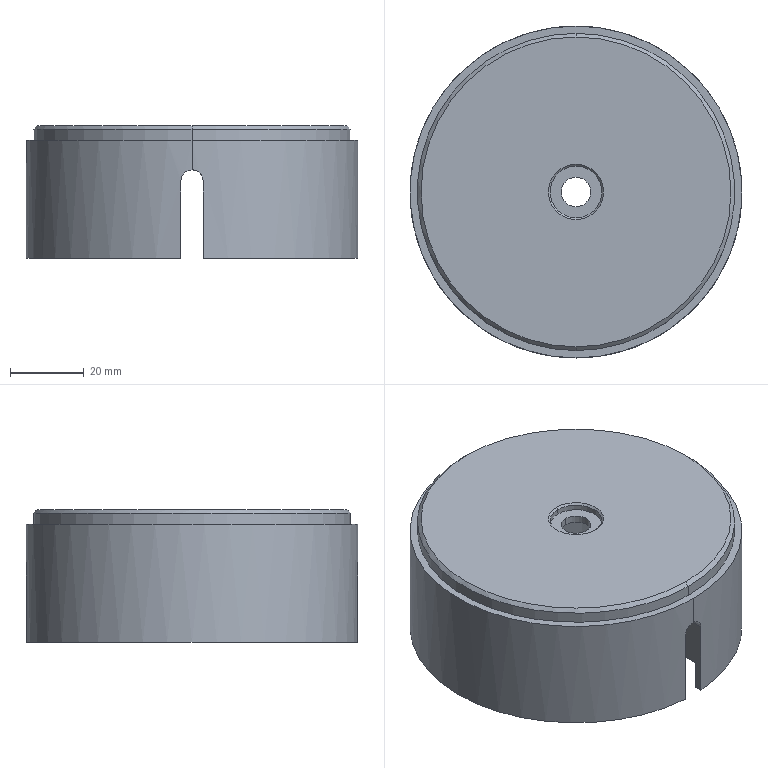Component | SolidWorks | GuideCover-1 | 1 solid | 32 faces | box 90 x 90 x 36 mm | volume 64020 mm3 | cylinder 14 | plane 12 | cone 4 | torus 2 | commonest cylinder face diameters 86 x4 14 x2 90 x2 8 x2 78 x2 6 x2
STEP:
#1=COLOUR_RGB('',0.7922,0.8196,0.9333);
#2=FILL_AREA_STYLE_COLOUR('',#1);
#3=FILL_AREA_STYLE('',(#2));
#4=SURFACE_STYLE_FILL_AREA(#3);
#5=SURFACE_SIDE_STYLE('',(#4));
#6=SURFACE_STYLE_USAGE(.BOTH.,#5);
#7=PRESENTATION_STYLE_ASSIGNMENT((#6));
#8=CARTESIAN_POINT('',(-0.6271,0.2087,2.579));
#9=VERTEX_POINT('',#8);
#10=CARTESIAN_POINT('',(-0.6271,-0.3425,2.579));
#11=VERTEX_POINT('',#10);
#12=CARTESIAN_POINT('',(-0.6271,-0.06694,2.579));
#13=DIRECTION('',(0.,0.,1.));
#14=DIRECTION('',(0.,-1.,0.));
#15=AXIS2_PLACEMENT_3D('',#12,#13,#14);
#16=CIRCLE('',#15,0.2756);
#17=EDGE_CURVE('',#9,#11,#16,.T.);
#18=ORIENTED_EDGE('',*,*,#17,.F.);
#19=CARTESIAN_POINT('',(-0.6271,0.2283,2.598));
#20=VERTEX_POINT('',#19);
#21=CARTESIAN_POINT('',(-0.6271,0.2087,2.579));
#22=DIRECTION('',(0.,0.7071,0.7071));
#23=VECTOR('',#22,39.37);
#24=LINE('',#21,#23);
#25=EDGE_CURVE('',#9,#20,#24,.T.);
#26=ORIENTED_EDGE('',*,*,#25,.T.);
#27=CARTESIAN_POINT('',(-0.6271,-0.3622,2.598));
#28=VERTEX_POINT('',#27);
#29=CARTESIAN_POINT('',(-0.6271,-0.06694,2.598));
#30=DIRECTION('',(0.,0.,-1.));
#31=DIRECTION('',(0.,-1.,0.));
#32=AXIS2_PLACEMENT_3D('',#29,#30,#31);
#33=CIRCLE('',#32,0.2953);
#34=EDGE_CURVE('',#28,#20,#33,.T.);
#35=ORIENTED_EDGE('',*,*,#34,.F.);
#36=CARTESIAN_POINT('',(-0.6271,-0.3425,2.579));
#37=DIRECTION('',(0.,-0.7071,0.7071));
#38=VECTOR('',#37,39.37);
#39=LINE('',#36,#38);
#40=EDGE_CURVE('',#11,#28,#39,.T.);
#41=ORIENTED_EDGE('',*,*,#40,.F.);
#42=EDGE_LOOP('',(#18,#26,#35,#41));
#43=FACE_OUTER_BOUND('',#42,.T.);
#44=CARTESIAN_POINT('',(-0.6271,-0.06694,2.579));
#45=DIRECTION('',(0.,0.,1.));
#46=DIRECTION('',(0.,-1.,0.));
#47=AXIS2_PLACEMENT_3D('',#44,#45,#46);
#48=CONICAL_SURFACE('',#47,0.2756,0.7854);
#49=ADVANCED_FACE('',(#43),#48,.F.);
#50=CARTESIAN_POINT('',(-0.6271,0.2087,2.52));
#51=VERTEX_POINT('',#50);
#52=CARTESIAN_POINT('',(-0.6271,-0.3425,2.52));
#53=VERTEX_POINT('',#52);
#54=CARTESIAN_POINT('',(-0.6271,-0.06694,2.52));
#55=DIRECTION('',(0.,0.,1.));
#56=DIRECTION('',(0.,-1.,0.));
#57=AXIS2_PLACEMENT_3D('',#54,#55,#56);
#58=CIRCLE('',#57,0.2756);
#59=EDGE_CURVE('',#51,#53,#58,.T.);
#60=ORIENTED_EDGE('',*,*,#59,.F.);
#61=CARTESIAN_POINT('',(-0.6271,0.2087,2.52));
#62=DIRECTION('',(0.,0.,1.));
#63=VECTOR('',#62,39.37);
#64=LINE('',#61,#63);
#65=EDGE_CURVE('',#51,#9,#64,.T.);
#66=ORIENTED_EDGE('',*,*,#65,.T.);
#67=ORIENTED_EDGE('',*,*,#17,.T.);
#68=CARTESIAN_POINT('',(-0.6271,-0.3425,2.52));
#69=DIRECTION('',(0.,0.,1.));
#70=VECTOR('',#69,39.37);
#71=LINE('',#68,#70);
#72=EDGE_CURVE('',#53,#11,#71,.T.);
#73=ORIENTED_EDGE('',*,*,#72,.F.);
#74=EDGE_LOOP('',(#60,#66,#67,#73));
#75=FACE_OUTER_BOUND('',#74,.T.);
#76=CARTESIAN_POINT('',(-0.6271,-0.06694,2.52));
#77=DIRECTION('',(0.,0.,1.));
#78=DIRECTION('',(0.,-1.,0.));
#79=AXIS2_PLACEMENT_3D('',#76,#77,#78);
#80=CYLINDRICAL_SURFACE('',#79,0.2756);
#81=ADVANCED_FACE('',(#75),#80,.F.);
#82=CARTESIAN_POINT('',(-0.6271,-1.72,2.598));
#83=VERTEX_POINT('',#82);
#84=CARTESIAN_POINT('',(-0.6271,1.587,2.598));
#85=VERTEX_POINT('',#84);
#86=CARTESIAN_POINT('',(-0.6271,-0.06694,2.598));
#87=DIRECTION('',(0.,0.,1.));
#88=DIRECTION('',(0.,-1.,0.));
#89=AXIS2_PLACEMENT_3D('',#86,#87,#88);
#90=CIRCLE('',#89,1.654);
#91=EDGE_CURVE('',#83,#85,#90,.T.);
#92=ORIENTED_EDGE('',*,*,#91,.F.);
#93=CARTESIAN_POINT('',(-0.6271,-1.76,2.559));
#94=VERTEX_POINT('',#93);
#95=CARTESIAN_POINT('',(-0.6271,-1.72,2.598));
#96=DIRECTION('',(0.,-0.7071,-0.7071));
#97=VECTOR('',#96,39.37);
#98=LINE('',#95,#97);
#99=EDGE_CURVE('',#83,#94,#98,.T.);
#100=ORIENTED_EDGE('',*,*,#99,.T.);
#101=CARTESIAN_POINT('',(-0.6271,1.626,2.559));
#102=VERTEX_POINT('',#101);
#103=CARTESIAN_POINT('',(-0.6271,-0.06694,2.559));
#104=DIRECTION('',(0.,0.,-1.));
#105=DIRECTION('',(0.,-1.,0.));
#106=AXIS2_PLACEMENT_3D('',#103,#104,#105);
#107=CIRCLE('',#106,1.693);
#108=EDGE_CURVE('',#102,#94,#107,.T.);
#109=ORIENTED_EDGE('',*,*,#108,.F.);
#110=CARTESIAN_POINT('',(-0.6271,1.587,2.598));
#111=DIRECTION('',(0.,0.7071,-0.7071));
#112=VECTOR('',#111,39.37);
#113=LINE('',#110,#112);
#114=EDGE_CURVE('',#85,#102,#113,.T.);
#115=ORIENTED_EDGE('',*,*,#114,.F.);
#116=EDGE_LOOP('',(#92,#100,#109,#115));
#117=FACE_OUTER_BOUND('',#116,.T.);
#118=CARTESIAN_POINT('',(-0.6271,-0.06694,2.598));
#119=DIRECTION('',(0.,0.,-1.));
#120=DIRECTION('',(0.,1.,0.));
#121=AXIS2_PLACEMENT_3D('',#118,#119,#120);
#122=CONICAL_SURFACE('',#121,1.654,0.7854);
#123=ADVANCED_FACE('',(#117),#122,.T.);
#124=CARTESIAN_POINT('',(-0.6271,1.468,2.362));
#125=VERTEX_POINT('',#124);
#126=CARTESIAN_POINT('',(-0.6271,-1.602,2.362));
#127=VERTEX_POINT('',#126);
#128=CARTESIAN_POINT('',(-0.6271,-0.06694,2.362));
#129=DIRECTION('',(0.,0.,1.));
#130=DIRECTION('',(0.,-1.,0.));
#131=AXIS2_PLACEMENT_3D('',#128,#129,#130);
#132=CIRCLE('',#131,1.535);
#133=EDGE_CURVE('',#125,#127,#132,.T.);
#134=ORIENTED_EDGE('',*,*,#133,.F.);
#135=CARTESIAN_POINT('',(-0.6271,1.39,2.441));
#136=VERTEX_POINT('',#135);
#137=CARTESIAN_POINT('',(-0.6271,1.39,2.362));
#138=DIRECTION('',(1.,-0.,0.));
#139=DIRECTION('',(0.,1.,0.));
#140=AXIS2_PLACEMENT_3D('',#137,#138,#139);
#141=CIRCLE('',#140,0.07874);
#142=EDGE_CURVE('',#125,#136,#141,.T.);
#143=ORIENTED_EDGE('',*,*,#142,.T.);
#144=CARTESIAN_POINT('',(-0.6271,-1.524,2.441));
#145=VERTEX_POINT('',#144);
#146=CARTESIAN_POINT('',(-0.6271,-0.06694,2.441));
#147=DIRECTION('',(0.,0.,-1.));
#148=DIRECTION('',(0.,-1.,0.));
#149=AXIS2_PLACEMENT_3D('',#146,#147,#148);
#150=CIRCLE('',#149,1.457);
#151=EDGE_CURVE('',#145,#136,#150,.T.);
#152=ORIENTED_EDGE('',*,*,#151,.F.);
#153=CARTESIAN_POINT('',(-0.6271,-1.524,2.362));
#154=DIRECTION('',(-1.,0.,0.));
#155=DIRECTION('',(0.,0.,1.));
#156=AXIS2_PLACEMENT_3D('',#153,#154,#155);
#157=CIRCLE('',#156,0.07874);
#158=EDGE_CURVE('',#127,#145,#157,.T.);
#159=ORIENTED_EDGE('',*,*,#158,.F.);
#160=EDGE_LOOP('',(#134,#143,#152,#159));
#161=FACE_OUTER_BOUND('',#160,.T.);
#162=CARTESIAN_POINT('',(-0.6271,-0.06694,2.362));
#163=DIRECTION('',(0.,0.,1.));
#164=DIRECTION('',(0.,-1.,0.));
#165=AXIS2_PLACEMENT_3D('',#162,#163,#164);
#166=TOROIDAL_SURFACE('',#165,1.457,0.07874);
#167=ADVANCED_FACE('',(#161),#166,.F.);
#168=CARTESIAN_POINT('',(-0.6271,-1.76,2.441));
#169=VERTEX_POINT('',#168);
#170=CARTESIAN_POINT('',(-0.6271,1.626,2.441));
#171=VERTEX_POINT('',#170);
#172=CARTESIAN_POINT('',(-0.6271,-0.06694,2.441));
#173=DIRECTION('',(0.,0.,1.));
#174=DIRECTION('',(0.,-1.,0.));
#175=AXIS2_PLACEMENT_3D('',#172,#173,#174);
#176=CIRCLE('',#175,1.693);
#177=EDGE_CURVE('',#169,#171,#176,.T.);
#178=ORIENTED_EDGE('',*,*,#177,.T.);
#179=CARTESIAN_POINT('',(-0.6271,1.626,3.116));
#180=DIRECTION('',(0.,0.,1.));
#181=VECTOR('',#180,39.37);
#182=LINE('',#179,#181);
#183=EDGE_CURVE('',#171,#102,#182,.T.);
#184=ORIENTED_EDGE('',*,*,#183,.T.);
#185=ORIENTED_EDGE('',*,*,#108,.T.);
#186=CARTESIAN_POINT('',(-0.6271,-1.76,3.116));
#187=DIRECTION('',(0.,0.,1.));
#188=VECTOR('',#187,39.37);
#189=LINE('',#186,#188);
#190=EDGE_CURVE('',#169,#94,#189,.T.);
#191=ORIENTED_EDGE('',*,*,#190,.F.);
#192=EDGE_LOOP('',(#178,#184,#185,#191));
#193=FACE_OUTER_BOUND('',#192,.T.);
#194=CARTESIAN_POINT('',(-0.6271,-0.06694,3.116));
#195=DIRECTION('',(0.,0.,1.));
#196=DIRECTION('',(0.,-1.,0.));
#197=AXIS2_PLACEMENT_3D('',#194,#195,#196);
#198=CYLINDRICAL_SURFACE('',#197,1.693);
#199=ADVANCED_FACE('',(#193),#198,.T.);
#200=CARTESIAN_POINT('',(-0.6271,-1.839,2.441));
#201=VERTEX_POINT('',#200);
#202=CARTESIAN_POINT('',(-0.6271,1.705,2.441));
#203=VERTEX_POINT('',#202);
#204=CARTESIAN_POINT('',(-0.6271,-0.06694,2.441));
#205=DIRECTION('',(0.,0.,1.));
#206=DIRECTION('',(0.,-1.,0.));
#207=AXIS2_PLACEMENT_3D('',#204,#205,#206);
#208=CIRCLE('',#207,1.772);
#209=EDGE_CURVE('',#201,#203,#208,.T.);
#210=ORIENTED_EDGE('',*,*,#209,.F.);
#211=CARTESIAN_POINT('',(-0.6271,-1.839,2.126));
#212=VERTEX_POINT('',#211);
#213=CARTESIAN_POINT('',(-0.6271,-1.839,2.598));
#214=DIRECTION('',(0.,0.,-1.));
#215=VECTOR('',#214,39.37);
#216=LINE('',#213,#215);
#217=EDGE_CURVE('',#201,#212,#216,.T.);
#218=ORIENTED_EDGE('',*,*,#217,.T.);
#219=CARTESIAN_POINT('',(-0.509,-1.835,2.008));
#220=VERTEX_POINT('',#219);
#221=CARTESIAN_POINT('',(-0.509,-1.835,2.008));
#222=CARTESIAN_POINT('',(-0.509,-1.835,2.023));
#223=CARTESIAN_POINT('',(-0.5121,-1.835,2.039));
#224=CARTESIAN_POINT('',(-0.521,-1.835,2.06));
#225=CARTESIAN_POINT('',(-0.5246,-1.836,2.067));
#226=CARTESIAN_POINT('',(-0.5333,-1.836,2.08));
#227=CARTESIAN_POINT('',(-0.5382,-1.836,2.086));
#228=CARTESIAN_POINT('',(-0.549,-1.837,2.097));
#229=CARTESIAN_POINT('',(-0.5551,-1.837,2.102));
#230=CARTESIAN_POINT('',(-0.568,-1.838,2.11));
#231=CARTESIAN_POINT('',(-0.5747,-1.838,2.114));
#232=CARTESIAN_POINT('',(-0.589,-1.838,2.12));
#233=CARTESIAN_POINT('',(-0.5965,-1.838,2.122));
#234=CARTESIAN_POINT('',(-0.6116,-1.839,2.125));
#235=CARTESIAN_POINT('',(-0.6193,-1.839,2.126));
#236=CARTESIAN_POINT('',(-0.6271,-1.839,2.126));
#237=B_SPLINE_CURVE_WITH_KNOTS('',3,(#221,#222,#223,#224,#225,#226,#227,#228,#229,#230,#231,#232,#233,#234,#235,#236),.UNSPECIFIED.,.F.,.F.,(4,2,2,2,2,2,2,4),(0.,0.001181,0.001772,0.002363,0.002954,0.003544,0.004135,0.004726),.UNSPECIFIED.);
#238=EDGE_CURVE('',#220,#212,#237,.T.);
#239=ORIENTED_EDGE('',*,*,#238,.F.);
#240=CARTESIAN_POINT('',(-0.509,-1.835,1.181));
#241=VERTEX_POINT('',#240);
#242=CARTESIAN_POINT('',(-0.509,-1.835,2.598));
#243=DIRECTION('',(0.,0.,-1.));
#244=VECTOR('',#243,39.37);
#245=LINE('',#242,#244);
#246=EDGE_CURVE('',#220,#241,#245,.T.);
#247=ORIENTED_EDGE('',*,*,#246,.T.);
#248=CARTESIAN_POINT('',(-0.509,1.701,1.181));
#249=VERTEX_POINT('',#248);
#250=CARTESIAN_POINT('',(-0.6271,-0.06694,1.181));
#251=DIRECTION('',(0.,0.,1.));
#252=DIRECTION('',(0.,-1.,0.));
#253=AXIS2_PLACEMENT_3D('',#250,#251,#252);
#254=CIRCLE('',#253,1.772);
#255=EDGE_CURVE('',#241,#249,#254,.T.);
#256=ORIENTED_EDGE('',*,*,#255,.T.);
#257=CARTESIAN_POINT('',(-0.509,1.701,2.008));
#258=VERTEX_POINT('',#257);
#259=CARTESIAN_POINT('',(-0.509,1.701,2.598));
#260=DIRECTION('',(0.,0.,1.));
#261=VECTOR('',#260,39.37);
#262=LINE('',#259,#261);
#263=EDGE_CURVE('',#249,#258,#262,.T.);
#264=ORIENTED_EDGE('',*,*,#263,.T.);
#265=CARTESIAN_POINT('',(-0.6271,1.705,2.126));
#266=VERTEX_POINT('',#265);
#267=CARTESIAN_POINT('',(-0.6271,1.705,2.126));
#268=CARTESIAN_POINT('',(-0.6115,1.705,2.126));
#269=CARTESIAN_POINT('',(-0.596,1.705,2.123));
#270=CARTESIAN_POINT('',(-0.5747,1.704,2.114));
#271=CARTESIAN_POINT('',(-0.5678,1.704,2.11));
#272=CARTESIAN_POINT('',(-0.5549,1.703,2.102));
#273=CARTESIAN_POINT('',(-0.549,1.703,2.097));
#274=CARTESIAN_POINT('',(-0.5381,1.702,2.086));
#275=CARTESIAN_POINT('',(-0.5331,1.702,2.08));
#276=CARTESIAN_POINT('',(-0.5246,1.702,2.067));
#277=CARTESIAN_POINT('',(-0.5209,1.702,2.06));
#278=CARTESIAN_POINT('',(-0.515,1.701,2.046));
#279=CARTESIAN_POINT('',(-0.5127,1.701,2.038));
#280=CARTESIAN_POINT('',(-0.5097,1.701,2.023));
#281=CARTESIAN_POINT('',(-0.509,1.701,2.016));
#282=CARTESIAN_POINT('',(-0.509,1.701,2.008));
#283=B_SPLINE_CURVE_WITH_KNOTS('',3,(#267,#268,#269,#270,#271,#272,#273,#274,#275,#276,#277,#278,#279,#280,#281,#282),.UNSPECIFIED.,.F.,.F.,(4,2,2,2,2,2,2,4),(0.004726,0.005907,0.006498,0.007089,0.00768,0.00827,0.008861,0.009452),.UNSPECIFIED.);
#284=EDGE_CURVE('',#266,#258,#283,.T.);
#285=ORIENTED_EDGE('',*,*,#284,.F.);
#286=CARTESIAN_POINT('',(-0.6271,1.705,2.598));
#287=DIRECTION('',(0.,0.,-1.));
#288=VECTOR('',#287,39.37);
#289=LINE('',#286,#288);
#290=EDGE_CURVE('',#203,#266,#289,.T.);
#291=ORIENTED_EDGE('',*,*,#290,.F.);
#292=EDGE_LOOP('',(#210,#218,#239,#247,#256,#264,#285,#291));
#293=FACE_OUTER_BOUND('',#292,.T.);
#294=CARTESIAN_POINT('',(-0.6271,-0.06694,2.598));
#295=DIRECTION('',(0.,0.,-1.));
#296=DIRECTION('',(0.,1.,0.));
#297=AXIS2_PLACEMENT_3D('',#294,#295,#296);
#298=CYLINDRICAL_SURFACE('',#297,1.772);
#299=ADVANCED_FACE('',(#293),#298,.T.);
#300=CARTESIAN_POINT('',(-0.6271,0.09054,2.441));
#301=VERTEX_POINT('',#300);
#302=CARTESIAN_POINT('',(-0.6271,-0.2244,2.441));
#303=VERTEX_POINT('',#302);
#304=CARTESIAN_POINT('',(-0.6271,-0.06694,2.441));
#305=DIRECTION('',(0.,0.,1.));
#306=DIRECTION('',(0.,-1.,0.));
#307=AXIS2_PLACEMENT_3D('',#304,#305,#306);
#308=CIRCLE('',#307,0.1575);
#309=EDGE_CURVE('',#301,#303,#308,.T.);
#310=ORIENTED_EDGE('',*,*,#309,.F.);
#311=CARTESIAN_POINT('',(-0.6271,0.09054,2.52));
#312=VERTEX_POINT('',#311);
#313=CARTESIAN_POINT('',(-0.6271,0.09054,2.441));
#314=DIRECTION('',(0.,0.,1.));
#315=VECTOR('',#314,39.37);
#316=LINE('',#313,#315);
#317=EDGE_CURVE('',#301,#312,#316,.T.);
#318=ORIENTED_EDGE('',*,*,#317,.T.);
#319=CARTESIAN_POINT('',(-0.6271,-0.2244,2.52));
#320=VERTEX_POINT('',#319);
#321=CARTESIAN_POINT('',(-0.6271,-0.06694,2.52));
#322=DIRECTION('',(0.,0.,-1.));
#323=DIRECTION('',(0.,-1.,0.));
#324=AXIS2_PLACEMENT_3D('',#321,#322,#323);
#325=CIRCLE('',#324,0.1575);
#326=EDGE_CURVE('',#320,#312,#325,.T.);
#327=ORIENTED_EDGE('',*,*,#326,.F.);
#328=CARTESIAN_POINT('',(-0.6271,-0.2244,2.441));
#329=DIRECTION('',(0.,0.,1.));
#330=VECTOR('',#329,39.37);
#331=LINE('',#328,#330);
#332=EDGE_CURVE('',#303,#320,#331,.T.);
#333=ORIENTED_EDGE('',*,*,#332,.F.);
#334=EDGE_LOOP('',(#310,#318,#327,#333));
#335=FACE_OUTER_BOUND('',#334,.T.);
#336=CARTESIAN_POINT('',(-0.6271,-0.06694,2.441));
#337=DIRECTION('',(0.,0.,1.));
#338=DIRECTION('',(0.,-1.,0.));
#339=AXIS2_PLACEMENT_3D('',#336,#337,#338);
#340=CYLINDRICAL_SURFACE('',#339,0.1575);
#341=ADVANCED_FACE('',(#335),#340,.F.);
#342=ORIENTED_EDGE('',*,*,#133,.T.);
#343=CARTESIAN_POINT('',(-0.6271,-1.602,2.126));
#344=VERTEX_POINT('',#343);
#345=CARTESIAN_POINT('',(-0.6271,-1.602,2.598));
#346=DIRECTION('',(0.,0.,-1.));
#347=VECTOR('',#346,39.37);
#348=LINE('',#345,#347);
#349=EDGE_CURVE('',#127,#344,#348,.T.);
#350=ORIENTED_EDGE('',*,*,#349,.T.);
#351=CARTESIAN_POINT('',(-0.7452,-1.598,2.008));
#352=VERTEX_POINT('',#351);
#353=CARTESIAN_POINT('',(-0.7452,-1.598,2.008));
#354=CARTESIAN_POINT('',(-0.7452,-1.598,2.023));
#355=CARTESIAN_POINT('',(-0.7421,-1.598,2.039));
#356=CARTESIAN_POINT('',(-0.7332,-1.599,2.06));
#357=CARTESIAN_POINT('',(-0.7295,-1.599,2.067));
#358=CARTESIAN_POINT('',(-0.7209,-1.6,2.08));
#359=CARTESIAN_POINT('',(-0.716,-1.6,2.086));
#360=CARTESIAN_POINT('',(-0.7051,-1.6,2.097));
#361=CARTESIAN_POINT('',(-0.6991,-1.601,2.102));
#362=CARTESIAN_POINT('',(-0.6862,-1.601,2.11));
#363=CARTESIAN_POINT('',(-0.6794,-1.601,2.114));
#364=CARTESIAN_POINT('',(-0.6651,-1.602,2.12));
#365=CARTESIAN_POINT('',(-0.6577,-1.602,2.122));
#366=CARTESIAN_POINT('',(-0.6426,-1.602,2.125));
#367=CARTESIAN_POINT('',(-0.6349,-1.602,2.126));
#368=CARTESIAN_POINT('',(-0.6271,-1.602,2.126));
#369=B_SPLINE_CURVE_WITH_KNOTS('',3,(#353,#354,#355,#356,#357,#358,#359,#360,#361,#362,#363,#364,#365,#366,#367,#368),.UNSPECIFIED.,.F.,.F.,(4,2,2,2,2,2,2,4),(0.,0.001182,0.001772,0.002363,0.002954,0.003545,0.004135,0.004726),.UNSPECIFIED.);
#370=EDGE_CURVE('',#352,#344,#369,.T.);
#371=ORIENTED_EDGE('',*,*,#370,.F.);
#372=CARTESIAN_POINT('',(-0.7452,-1.598,1.496));
#373=VERTEX_POINT('',#372);
#374=CARTESIAN_POINT('',(-0.7452,-1.598,2.598));
#375=DIRECTION('',(0.,0.,1.));
#376=VECTOR('',#375,39.37);
#377=LINE('',#374,#376);
#378=EDGE_CURVE('',#373,#352,#377,.T.);
#379=ORIENTED_EDGE('',*,*,#378,.F.);
#380=CARTESIAN_POINT('',(-0.7452,1.464,1.496));
#381=VERTEX_POINT('',#380);
#382=CARTESIAN_POINT('',(-0.6271,-0.06694,1.496));
#383=DIRECTION('',(0.,0.,-1.));
#384=DIRECTION('',(0.,1.,0.));
#385=AXIS2_PLACEMENT_3D('',#382,#383,#384);
#386=CIRCLE('',#385,1.535);
#387=EDGE_CURVE('',#373,#381,#386,.T.);
#388=ORIENTED_EDGE('',*,*,#387,.T.);
#389=CARTESIAN_POINT('',(-0.7452,1.464,2.008));
#390=VERTEX_POINT('',#389);
#391=CARTESIAN_POINT('',(-0.7452,1.464,2.598));
#392=DIRECTION('',(0.,0.,-1.));
#393=VECTOR('',#392,39.37);
#394=LINE('',#391,#393);
#395=EDGE_CURVE('',#390,#381,#394,.T.);
#396=ORIENTED_EDGE('',*,*,#395,.F.);
#397=CARTESIAN_POINT('',(-0.6271,1.468,2.126));
#398=VERTEX_POINT('',#397);
#399=CARTESIAN_POINT('',(-0.6271,1.468,2.126));
#400=CARTESIAN_POINT('',(-0.6427,1.468,2.126));
#401=CARTESIAN_POINT('',(-0.6582,1.468,2.123));
#402=CARTESIAN_POINT('',(-0.6795,1.468,2.114));
#403=CARTESIAN_POINT('',(-0.6864,1.467,2.11));
#404=CARTESIAN_POINT('',(-0.6993,1.467,2.102));
#405=CARTESIAN_POINT('',(-0.7052,1.467,2.097));
#406=CARTESIAN_POINT('',(-0.7161,1.466,2.086));
#407=CARTESIAN_POINT('',(-0.7211,1.466,2.08));
#408=CARTESIAN_POINT('',(-0.7296,1.465,2.067));
#409=CARTESIAN_POINT('',(-0.7332,1.465,2.06));
#410=CARTESIAN_POINT('',(-0.7392,1.464,2.046));
#411=CARTESIAN_POINT('',(-0.7414,1.464,2.038));
#412=CARTESIAN_POINT('',(-0.7444,1.464,2.023));
#413=CARTESIAN_POINT('',(-0.7452,1.464,2.016));
#414=CARTESIAN_POINT('',(-0.7452,1.464,2.008));
#415=B_SPLINE_CURVE_WITH_KNOTS('',3,(#399,#400,#401,#402,#403,#404,#405,#406,#407,#408,#409,#410,#411,#412,#413,#414),.UNSPECIFIED.,.F.,.F.,(4,2,2,2,2,2,2,4),(0.004726,0.005908,0.006499,0.007089,0.00768,0.008271,0.008862,0.009452),.UNSPECIFIED.);
#416=EDGE_CURVE('',#398,#390,#415,.T.);
#417=ORIENTED_EDGE('',*,*,#416,.F.);
#418=CARTESIAN_POINT('',(-0.6271,1.468,2.598));
#419=DIRECTION('',(0.,0.,-1.));
#420=VECTOR('',#419,39.37);
#421=LINE('',#418,#420);
#422=EDGE_CURVE('',#125,#398,#421,.T.);
#423=ORIENTED_EDGE('',*,*,#422,.F.);
#424=EDGE_LOOP('',(#342,#350,#371,#379,#388,#396,#417,#423));
#425=FACE_OUTER_BOUND('',#424,.T.);
#426=CARTESIAN_POINT('',(-0.6271,-0.06694,2.598));
#427=DIRECTION('',(0.,0.,-1.));
#428=DIRECTION('',(0.,1.,0.));
#429=AXIS2_PLACEMENT_3D('',#426,#427,#428);
#430=CYLINDRICAL_SURFACE('',#429,1.535);
#431=ADVANCED_FACE('',(#425),#430,.F.);
#432=ORIENTED_EDGE('',*,*,#349,.F.);
#433=CARTESIAN_POINT('',(-0.6271,-0.06694,2.362));
#434=DIRECTION('',(0.,0.,1.));
#435=DIRECTION('',(0.,-1.,0.));
#436=AXIS2_PLACEMENT_3D('',#433,#434,#435);
#437=CIRCLE('',#436,1.535);
#438=EDGE_CURVE('',#127,#125,#437,.T.);
#439=ORIENTED_EDGE('',*,*,#438,.T.);
#440=ORIENTED_EDGE('',*,*,#422,.T.);
#441=CARTESIAN_POINT('',(-0.509,1.464,2.008));
#442=VERTEX_POINT('',#441);
#443=CARTESIAN_POINT('',(-0.509,1.464,2.008));
#444=CARTESIAN_POINT('',(-0.509,1.464,2.023));
#445=CARTESIAN_POINT('',(-0.5121,1.464,2.039));
#446=CARTESIAN_POINT('',(-0.521,1.465,2.06));
#447=CARTESIAN_POINT('',(-0.5246,1.465,2.067));
#448=CARTESIAN_POINT('',(-0.5333,1.466,2.08));
#449=CARTESIAN_POINT('',(-0.5382,1.466,2.086));
#450=CARTESIAN_POINT('',(-0.549,1.467,2.097));
#451=CARTESIAN_POINT('',(-0.5551,1.467,2.102));
#452=CARTESIAN_POINT('',(-0.568,1.467,2.11));
#453=CARTESIAN_POINT('',(-0.5747,1.468,2.114));
#454=CARTESIAN_POINT('',(-0.589,1.468,2.12));
#455=CARTESIAN_POINT('',(-0.5965,1.468,2.122));
#456=CARTESIAN_POINT('',(-0.6116,1.468,2.125));
#457=CARTESIAN_POINT('',(-0.6193,1.468,2.126));
#458=CARTESIAN_POINT('',(-0.6271,1.468,2.126));
#459=B_SPLINE_CURVE_WITH_KNOTS('',3,(#443,#444,#445,#446,#447,#448,#449,#450,#451,#452,#453,#454,#455,#456,#457,#458),.UNSPECIFIED.,.F.,.F.,(4,2,2,2,2,2,2,4),(0.,0.001182,0.001772,0.002363,0.002954,0.003545,0.004135,0.004726),.UNSPECIFIED.);
#460=EDGE_CURVE('',#442,#398,#459,.T.);
#461=ORIENTED_EDGE('',*,*,#460,.F.);
#462=CARTESIAN_POINT('',(-0.509,1.464,1.496));
#463=VERTEX_POINT('',#462);
#464=CARTESIAN_POINT('',(-0.509,1.464,2.598));
#465=DIRECTION('',(0.,0.,1.));
#466=VECTOR('',#465,39.37);
#467=LINE('',#464,#466);
#468=EDGE_CURVE('',#463,#442,#467,.T.);
#469=ORIENTED_EDGE('',*,*,#468,.F.);
#470=CARTESIAN_POINT('',(-0.509,-1.598,1.496));
#471=VERTEX_POINT('',#470);
#472=CARTESIAN_POINT('',(-0.6271,-0.06694,1.496));
#473=DIRECTION('',(0.,0.,-1.));
#474=DIRECTION('',(0.,1.,0.));
#475=AXIS2_PLACEMENT_3D('',#472,#473,#474);
#476=CIRCLE('',#475,1.535);
#477=EDGE_CURVE('',#463,#471,#476,.T.);
#478=ORIENTED_EDGE('',*,*,#477,.T.);
#479=CARTESIAN_POINT('',(-0.509,-1.598,2.008));
#480=VERTEX_POINT('',#479);
#481=CARTESIAN_POINT('',(-0.509,-1.598,2.598));
#482=DIRECTION('',(0.,0.,-1.));
#483=VECTOR('',#482,39.37);
#484=LINE('',#481,#483);
#485=EDGE_CURVE('',#480,#471,#484,.T.);
#486=ORIENTED_EDGE('',*,*,#485,.F.);
#487=CARTESIAN_POINT('',(-0.6271,-1.602,2.126));
#488=CARTESIAN_POINT('',(-0.6115,-1.602,2.126));
#489=CARTESIAN_POINT('',(-0.596,-1.602,2.123));
#490=CARTESIAN_POINT('',(-0.5747,-1.601,2.114));
#491=CARTESIAN_POINT('',(-0.5678,-1.601,2.11));
#492=CARTESIAN_POINT('',(-0.5549,-1.601,2.102));
#493=CARTESIAN_POINT('',(-0.549,-1.6,2.097));
#494=CARTESIAN_POINT('',(-0.5381,-1.6,2.086));
#495=CARTESIAN_POINT('',(-0.5331,-1.599,2.08));
#496=CARTESIAN_POINT('',(-0.5246,-1.599,2.067));
#497=CARTESIAN_POINT('',(-0.5209,-1.599,2.06));
#498=CARTESIAN_POINT('',(-0.515,-1.598,2.046));
#499=CARTESIAN_POINT('',(-0.5127,-1.598,2.038));
#500=CARTESIAN_POINT('',(-0.5097,-1.598,2.023));
#501=CARTESIAN_POINT('',(-0.509,-1.598,2.016));
#502=CARTESIAN_POINT('',(-0.509,-1.598,2.008));
#503=B_SPLINE_CURVE_WITH_KNOTS('',3,(#487,#488,#489,#490,#491,#492,#493,#494,#495,#496,#497,#498,#499,#500,#501,#502),.UNSPECIFIED.,.F.,.F.,(4,2,2,2,2,2,2,4),(0.004726,0.005908,0.006499,0.007089,0.00768,0.008271,0.008862,0.009452),.UNSPECIFIED.);
#504=EDGE_CURVE('',#344,#480,#503,.T.);
#505=ORIENTED_EDGE('',*,*,#504,.F.);
#506=EDGE_LOOP('',(#432,#439,#440,#461,#469,#478,#486,#505));
#507=FACE_OUTER_BOUND('',#506,.T.);
#508=CARTESIAN_POINT('',(-0.6271,-0.06694,2.598));
#509=DIRECTION('',(0.,0.,-1.));
#510=DIRECTION('',(0.,1.,0.));
#511=AXIS2_PLACEMENT_3D('',#508,#509,#510);
#512=CYLINDRICAL_SURFACE('',#511,1.535);
#513=ADVANCED_FACE('',(#507),#512,.F.);
#514=ORIENTED_EDGE('',*,*,#317,.F.);
#515=CARTESIAN_POINT('',(-0.6271,-0.06694,2.441));
#516=DIRECTION('',(0.,0.,1.));
#517=DIRECTION('',(0.,-1.,0.));
#518=AXIS2_PLACEMENT_3D('',#515,#516,#517);
#519=CIRCLE('',#518,0.1575);
#520=EDGE_CURVE('',#303,#301,#519,.T.);
#521=ORIENTED_EDGE('',*,*,#520,.F.);
#522=ORIENTED_EDGE('',*,*,#332,.T.);
#523=CARTESIAN_POINT('',(-0.6271,-0.06694,2.52));
#524=DIRECTION('',(0.,0.,-1.));
#525=DIRECTION('',(0.,-1.,0.));
#526=AXIS2_PLACEMENT_3D('',#523,#524,#525);
#527=CIRCLE('',#526,0.1575);
#528=EDGE_CURVE('',#312,#320,#527,.T.);
#529=ORIENTED_EDGE('',*,*,#528,.F.);
#530=EDGE_LOOP('',(#514,#521,#522,#529));
#531=FACE_OUTER_BOUND('',#530,.T.);
#532=CARTESIAN_POINT('',(-0.6271,-0.06694,2.441));
#533=DIRECTION('',(0.,0.,1.));
#534=DIRECTION('',(0.,-1.,0.));
#535=AXIS2_PLACEMENT_3D('',#532,#533,#534);
#536=CYLINDRICAL_SURFACE('',#535,0.1575);
#537=ADVANCED_FACE('',(#531),#536,.F.);
#538=CARTESIAN_POINT('',(-0.509,1.464,2.008));
#539=DIRECTION('',(0.,1.,0.));
#540=VECTOR('',#539,39.37);
#541=LINE('',#538,#540);
#542=EDGE_CURVE('',#442,#258,#541,.T.);
#543=ORIENTED_EDGE('',*,*,#542,.F.);
#544=ORIENTED_EDGE('',*,*,#460,.T.);
#545=ORIENTED_EDGE('',*,*,#416,.T.);
#546=CARTESIAN_POINT('',(-0.7452,1.701,2.008));
#547=VERTEX_POINT('',#546);
#548=CARTESIAN_POINT('',(-0.7452,1.464,2.008));
#549=DIRECTION('',(0.,-1.,0.));
#550=VECTOR('',#549,39.37);
#551=LINE('',#548,#550);
#552=EDGE_CURVE('',#547,#390,#551,.T.);
#553=ORIENTED_EDGE('',*,*,#552,.F.);
#554=CARTESIAN_POINT('',(-0.7452,1.701,2.008));
#555=CARTESIAN_POINT('',(-0.7452,1.701,2.023));
#556=CARTESIAN_POINT('',(-0.7421,1.701,2.039));
#557=CARTESIAN_POINT('',(-0.7332,1.702,2.06));
#558=CARTESIAN_POINT('',(-0.7295,1.702,2.067));
#559=CARTESIAN_POINT('',(-0.7209,1.702,2.08));
#560=CARTESIAN_POINT('',(-0.716,1.702,2.086));
#561=CARTESIAN_POINT('',(-0.7051,1.703,2.097));
#562=CARTESIAN_POINT('',(-0.6991,1.703,2.102));
#563=CARTESIAN_POINT('',(-0.6862,1.704,2.11));
#564=CARTESIAN_POINT('',(-0.6794,1.704,2.114));
#565=CARTESIAN_POINT('',(-0.6651,1.704,2.12));
#566=CARTESIAN_POINT('',(-0.6576,1.704,2.122));
#567=CARTESIAN_POINT('',(-0.6426,1.705,2.125));
#568=CARTESIAN_POINT('',(-0.6349,1.705,2.126));
#569=CARTESIAN_POINT('',(-0.6271,1.705,2.126));
#570=B_SPLINE_CURVE_WITH_KNOTS('',3,(#554,#555,#556,#557,#558,#559,#560,#561,#562,#563,#564,#565,#566,#567,#568,#569),.UNSPECIFIED.,.F.,.F.,(4,2,2,2,2,2,2,4),(0.,0.001181,0.001772,0.002363,0.002954,0.003544,0.004135,0.004726),.UNSPECIFIED.);
#571=EDGE_CURVE('',#547,#266,#570,.T.);
#572=ORIENTED_EDGE('',*,*,#571,.T.);
#573=ORIENTED_EDGE('',*,*,#284,.T.);
#574=EDGE_LOOP('',(#543,#544,#545,#553,#572,#573));
#575=FACE_OUTER_BOUND('',#574,.T.);
#576=CARTESIAN_POINT('',(-0.6271,1.464,2.008));
#577=DIRECTION('',(0.,-1.,0.));
#578=DIRECTION('',(1.,0.,0.));
#579=AXIS2_PLACEMENT_3D('',#576,#577,#578);
#580=CYLINDRICAL_SURFACE('',#579,0.1181);
#581=ADVANCED_FACE('',(#575),#580,.F.);
#582=CARTESIAN_POINT('',(-0.7452,-1.835,2.008));
#583=VERTEX_POINT('',#582);
#584=CARTESIAN_POINT('',(-0.7452,-1.598,2.008));
#585=DIRECTION('',(0.,-1.,0.));
#586=VECTOR('',#585,39.37);
#587=LINE('',#584,#586);
#588=EDGE_CURVE('',#352,#583,#587,.T.);
#589=ORIENTED_EDGE('',*,*,#588,.F.);
#590=ORIENTED_EDGE('',*,*,#370,.T.);
#591=ORIENTED_EDGE('',*,*,#504,.T.);
#592=CARTESIAN_POINT('',(-0.509,-1.598,2.008));
#593=DIRECTION('',(0.,1.,0.));
#594=VECTOR('',#593,39.37);
#595=LINE('',#592,#594);
#596=EDGE_CURVE('',#220,#480,#595,.T.);
#597=ORIENTED_EDGE('',*,*,#596,.F.);
#598=ORIENTED_EDGE('',*,*,#238,.T.);
#599=CARTESIAN_POINT('',(-0.6271,-1.839,2.126));
#600=CARTESIAN_POINT('',(-0.6427,-1.839,2.126));
#601=CARTESIAN_POINT('',(-0.6582,-1.838,2.123));
#602=CARTESIAN_POINT('',(-0.6795,-1.838,2.114));
#603=CARTESIAN_POINT('',(-0.6864,-1.838,2.11));
#604=CARTESIAN_POINT('',(-0.6993,-1.837,2.102));
#605=CARTESIAN_POINT('',(-0.7052,-1.837,2.097));
#606=CARTESIAN_POINT('',(-0.7161,-1.836,2.086));
#607=CARTESIAN_POINT('',(-0.7211,-1.836,2.08));
#608=CARTESIAN_POINT('',(-0.7296,-1.836,2.067));
#609=CARTESIAN_POINT('',(-0.7332,-1.835,2.06));
#610=CARTESIAN_POINT('',(-0.7392,-1.835,2.046));
#611=CARTESIAN_POINT('',(-0.7414,-1.835,2.038));
#612=CARTESIAN_POINT('',(-0.7444,-1.835,2.023));
#613=CARTESIAN_POINT('',(-0.7452,-1.835,2.016));
#614=CARTESIAN_POINT('',(-0.7452,-1.835,2.008));
#615=B_SPLINE_CURVE_WITH_KNOTS('',3,(#599,#600,#601,#602,#603,#604,#605,#606,#607,#608,#609,#610,#611,#612,#613,#614),.UNSPECIFIED.,.F.,.F.,(4,2,2,2,2,2,2,4),(0.004726,0.005907,0.006498,0.007089,0.00768,0.00827,0.008861,0.009452),.UNSPECIFIED.);
#616=EDGE_CURVE('',#212,#583,#615,.T.);
#617=ORIENTED_EDGE('',*,*,#616,.T.);
#618=EDGE_LOOP('',(#589,#590,#591,#597,#598,#617));
#619=FACE_OUTER_BOUND('',#618,.T.);
#620=CARTESIAN_POINT('',(-0.6271,-1.598,2.008));
#621=DIRECTION('',(0.,-1.,0.));
#622=DIRECTION('',(1.,0.,0.));
#623=AXIS2_PLACEMENT_3D('',#620,#621,#622);
#624=CYLINDRICAL_SURFACE('',#623,0.1181);
#625=ADVANCED_FACE('',(#619),#624,.F.);
#626=ORIENTED_EDGE('',*,*,#255,.F.);
#627=CARTESIAN_POINT('',(-0.509,-1.756,1.181));
#628=VERTEX_POINT('',#627);
#629=CARTESIAN_POINT('',(-0.509,-0.06694,1.181));
#630=DIRECTION('',(0.,1.,0.));
#631=VECTOR('',#630,39.37);
#632=LINE('',#629,#631);
#633=EDGE_CURVE('',#241,#628,#632,.T.);
#634=ORIENTED_EDGE('',*,*,#633,.T.);
#635=CARTESIAN_POINT('',(-0.509,1.622,1.181));
#636=VERTEX_POINT('',#635);
#637=CARTESIAN_POINT('',(-0.6271,-0.06694,1.181));
#638=DIRECTION('',(0.,0.,1.));
#639=DIRECTION('',(0.,-1.,0.));
#640=AXIS2_PLACEMENT_3D('',#637,#638,#639);
#641=CIRCLE('',#640,1.693);
#642=EDGE_CURVE('',#628,#636,#641,.T.);
#643=ORIENTED_EDGE('',*,*,#642,.T.);
#644=CARTESIAN_POINT('',(-0.509,-0.06694,1.181));
#645=DIRECTION('',(0.,1.,0.));
#646=VECTOR('',#645,39.37);
#647=LINE('',#644,#646);
#648=EDGE_CURVE('',#636,#249,#647,.T.);
#649=ORIENTED_EDGE('',*,*,#648,.T.);
#650=EDGE_LOOP('',(#626,#634,#643,#649));
#651=FACE_OUTER_BOUND('',#650,.T.);
#652=CARTESIAN_POINT('',(-0.6271,-0.06694,1.181));
#653=DIRECTION('',(0.,0.,1.));
#654=DIRECTION('',(0.,-1.,0.));
#655=AXIS2_PLACEMENT_3D('',#652,#653,#654);
#656=PLANE('',#655);
#657=ADVANCED_FACE('',(#651),#656,.F.);
#658=CARTESIAN_POINT('',(-0.509,-1.756,1.496));
#659=VERTEX_POINT('',#658);
#660=CARTESIAN_POINT('',(-0.509,-1.756,3.14));
#661=DIRECTION('',(0.,0.,1.));
#662=VECTOR('',#661,39.37);
#663=LINE('',#660,#662);
#664=EDGE_CURVE('',#628,#659,#663,.T.);
#665=ORIENTED_EDGE('',*,*,#664,.T.);
#666=CARTESIAN_POINT('',(-0.509,1.622,1.496));
#667=VERTEX_POINT('',#666);
#668=CARTESIAN_POINT('',(-0.6271,-0.06694,1.496));
#669=DIRECTION('',(0.,0.,-1.));
#670=DIRECTION('',(0.,1.,0.));
#671=AXIS2_PLACEMENT_3D('',#668,#669,#670);
#672=CIRCLE('',#671,1.693);
#673=EDGE_CURVE('',#667,#659,#672,.T.);
#674=ORIENTED_EDGE('',*,*,#673,.F.);
#675=CARTESIAN_POINT('',(-0.509,1.622,3.14));
#676=DIRECTION('',(0.,0.,-1.));
#677=VECTOR('',#676,39.37);
#678=LINE('',#675,#677);
#679=EDGE_CURVE('',#667,#636,#678,.T.);
#680=ORIENTED_EDGE('',*,*,#679,.T.);
#681=ORIENTED_EDGE('',*,*,#642,.F.);
#682=EDGE_LOOP('',(#665,#674,#680,#681));
#683=FACE_OUTER_BOUND('',#682,.T.);
#684=CARTESIAN_POINT('',(-0.6271,-0.06694,3.14));
#685=DIRECTION('',(0.,0.,1.));
#686=DIRECTION('',(0.,-1.,0.));
#687=AXIS2_PLACEMENT_3D('',#684,#685,#686);
#688=CYLINDRICAL_SURFACE('',#687,1.693);
#689=ADVANCED_FACE('',(#683),#688,.F.);
#690=ORIENTED_EDGE('',*,*,#34,.T.);
#691=CARTESIAN_POINT('',(-0.6271,-0.06694,2.598));
#692=DIRECTION('',(0.,0.,-1.));
#693=DIRECTION('',(0.,-1.,0.));
#694=AXIS2_PLACEMENT_3D('',#691,#692,#693);
#695=CIRCLE('',#694,0.2953);
#696=EDGE_CURVE('',#20,#28,#695,.T.);
#697=ORIENTED_EDGE('',*,*,#696,.T.);
#698=EDGE_LOOP('',(#690,#697));
#699=FACE_BOUND('',#698,.T.);
#700=CARTESIAN_POINT('',(-0.6271,-0.06694,2.598));
#701=DIRECTION('',(0.,0.,1.));
#702=DIRECTION('',(0.,-1.,0.));
#703=AXIS2_PLACEMENT_3D('',#700,#701,#702);
#704=CIRCLE('',#703,1.654);
#705=EDGE_CURVE('',#85,#83,#704,.T.);
#706=ORIENTED_EDGE('',*,*,#705,.T.);
#707=ORIENTED_EDGE('',*,*,#91,.T.);
#708=EDGE_LOOP('',(#706,#707));
#709=FACE_OUTER_BOUND('',#708,.T.);
#710=CARTESIAN_POINT('',(-0.6271,-0.06694,2.598));
#711=DIRECTION('',(0.,0.,1.));
#712=DIRECTION('',(0.,-1.,0.));
#713=AXIS2_PLACEMENT_3D('',#710,#711,#712);
#714=PLANE('',#713);
#715=ADVANCED_FACE('',(#699,#709),#714,.T.);
#716=CARTESIAN_POINT('',(-0.7452,1.701,1.181));
#717=VERTEX_POINT('',#716);
#718=CARTESIAN_POINT('',(-0.7452,-1.835,1.181));
#719=VERTEX_POINT('',#718);
#720=CARTESIAN_POINT('',(-0.6271,-0.06694,1.181));
#721=DIRECTION('',(0.,0.,1.));
#722=DIRECTION('',(0.,-1.,0.));
#723=AXIS2_PLACEMENT_3D('',#720,#721,#722);
#724=CIRCLE('',#723,1.772);
#725=EDGE_CURVE('',#717,#719,#724,.T.);
#726=ORIENTED_EDGE('',*,*,#725,.F.);
#727=CARTESIAN_POINT('',(-0.7452,1.622,1.181));
#728=VERTEX_POINT('',#727);
#729=CARTESIAN_POINT('',(-0.7452,-0.06694,1.181));
#730=DIRECTION('',(0.,-1.,0.));
#731=VECTOR('',#730,39.37);
#732=LINE('',#729,#731);
#733=EDGE_CURVE('',#717,#728,#732,.T.);
#734=ORIENTED_EDGE('',*,*,#733,.T.);
#735=CARTESIAN_POINT('',(-0.7452,-1.756,1.181));
#736=VERTEX_POINT('',#735);
#737=CARTESIAN_POINT('',(-0.6271,-0.06694,1.181));
#738=DIRECTION('',(0.,0.,1.));
#739=DIRECTION('',(0.,-1.,0.));
#740=AXIS2_PLACEMENT_3D('',#737,#738,#739);
#741=CIRCLE('',#740,1.693);
#742=EDGE_CURVE('',#728,#736,#741,.T.);
#743=ORIENTED_EDGE('',*,*,#742,.T.);
#744=CARTESIAN_POINT('',(-0.7452,-0.06694,1.181));
#745=DIRECTION('',(0.,-1.,0.));
#746=VECTOR('',#745,39.37);
#747=LINE('',#744,#746);
#748=EDGE_CURVE('',#736,#719,#747,.T.);
#749=ORIENTED_EDGE('',*,*,#748,.T.);
#750=EDGE_LOOP('',(#726,#734,#743,#749));
#751=FACE_OUTER_BOUND('',#750,.T.);
#752=CARTESIAN_POINT('',(-0.6271,-0.06694,1.181));
#753=DIRECTION('',(0.,0.,1.));
#754=DIRECTION('',(0.,-1.,0.));
#755=AXIS2_PLACEMENT_3D('',#752,#753,#754);
#756=PLANE('',#755);
#757=ADVANCED_FACE('',(#751),#756,.F.);
#758=ORIENTED_EDGE('',*,*,#217,.F.);
#759=CARTESIAN_POINT('',(-0.6271,-0.06694,2.441));
#760=DIRECTION('',(0.,0.,1.));
#761=DIRECTION('',(0.,-1.,0.));
#762=AXIS2_PLACEMENT_3D('',#759,#760,#761);
#763=CIRCLE('',#762,1.772);
#764=EDGE_CURVE('',#203,#201,#763,.T.);
#765=ORIENTED_EDGE('',*,*,#764,.F.);
#766=ORIENTED_EDGE('',*,*,#290,.T.);
#767=ORIENTED_EDGE('',*,*,#571,.F.);
#768=CARTESIAN_POINT('',(-0.7452,1.701,2.598));
#769=DIRECTION('',(0.,0.,-1.));
#770=VECTOR('',#769,39.37);
#771=LINE('',#768,#770);
#772=EDGE_CURVE('',#547,#717,#771,.T.);
#773=ORIENTED_EDGE('',*,*,#772,.T.);
#774=ORIENTED_EDGE('',*,*,#725,.T.);
#775=CARTESIAN_POINT('',(-0.7452,-1.835,2.598));
#776=DIRECTION('',(0.,0.,1.));
#777=VECTOR('',#776,39.37);
#778=LINE('',#775,#777);
#779=EDGE_CURVE('',#719,#583,#778,.T.);
#780=ORIENTED_EDGE('',*,*,#779,.T.);
#781=ORIENTED_EDGE('',*,*,#616,.F.);
#782=EDGE_LOOP('',(#758,#765,#766,#767,#773,#774,#780,#781));
#783=FACE_OUTER_BOUND('',#782,.T.);
#784=CARTESIAN_POINT('',(-0.6271,-0.06694,2.598));
#785=DIRECTION('',(0.,0.,-1.));
#786=DIRECTION('',(0.,1.,0.));
#787=AXIS2_PLACEMENT_3D('',#784,#785,#786);
#788=CYLINDRICAL_SURFACE('',#787,1.772);
#789=ADVANCED_FACE('',(#783),#788,.T.);
#790=CARTESIAN_POINT('',(-0.7452,1.622,1.496));
#791=VERTEX_POINT('',#790);
#792=CARTESIAN_POINT('',(-0.7452,1.622,3.14));
#793=DIRECTION('',(0.,0.,1.));
#794=VECTOR('',#793,39.37);
#795=LINE('',#792,#794);
#796=EDGE_CURVE('',#728,#791,#795,.T.);
#797=ORIENTED_EDGE('',*,*,#796,.T.);
#798=CARTESIAN_POINT('',(-0.7452,-1.756,1.496));
#799=VERTEX_POINT('',#798);
#800=CARTESIAN_POINT('',(-0.6271,-0.06694,1.496));
#801=DIRECTION('',(0.,0.,-1.));
#802=DIRECTION('',(0.,1.,0.));
#803=AXIS2_PLACEMENT_3D('',#800,#801,#802);
#804=CIRCLE('',#803,1.693);
#805=EDGE_CURVE('',#799,#791,#804,.T.);
#806=ORIENTED_EDGE('',*,*,#805,.F.);
#807=CARTESIAN_POINT('',(-0.7452,-1.756,3.14));
#808=DIRECTION('',(0.,0.,-1.));
#809=VECTOR('',#808,39.37);
#810=LINE('',#807,#809);
#811=EDGE_CURVE('',#799,#736,#810,.T.);
#812=ORIENTED_EDGE('',*,*,#811,.T.);
#813=ORIENTED_EDGE('',*,*,#742,.F.);
#814=EDGE_LOOP('',(#797,#806,#812,#813));
#815=FACE_OUTER_BOUND('',#814,.T.);
#816=CARTESIAN_POINT('',(-0.6271,-0.06694,3.14));
#817=DIRECTION('',(0.,0.,1.));
#818=DIRECTION('',(0.,-1.,0.));
#819=AXIS2_PLACEMENT_3D('',#816,#817,#818);
#820=CYLINDRICAL_SURFACE('',#819,1.693);
#821=ADVANCED_FACE('',(#815),#820,.F.);
#822=ORIENTED_EDGE('',*,*,#151,.T.);
#823=CARTESIAN_POINT('',(-0.6271,-0.06694,2.441));
#824=DIRECTION('',(0.,0.,-1.));
#825=DIRECTION('',(0.,-1.,0.));
#826=AXIS2_PLACEMENT_3D('',#823,#824,#825);
#827=CIRCLE('',#826,1.457);
#828=EDGE_CURVE('',#136,#145,#827,.T.);
#829=ORIENTED_EDGE('',*,*,#828,.T.);
#830=EDGE_LOOP('',(#822,#829));
#831=FACE_OUTER_BOUND('',#830,.T.);
#832=ORIENTED_EDGE('',*,*,#520,.T.);
#833=ORIENTED_EDGE('',*,*,#309,.T.);
#834=EDGE_LOOP('',(#832,#833));
#835=FACE_BOUND('',#834,.T.);
#836=CARTESIAN_POINT('',(-0.6271,-0.06694,2.441));
#837=DIRECTION('',(0.,0.,1.));
#838=DIRECTION('',(0.,-1.,0.));
#839=AXIS2_PLACEMENT_3D('',#836,#837,#838);
#840=PLANE('',#839);
#841=ADVANCED_FACE('',(#831,#835),#840,.F.);
#842=ORIENTED_EDGE('',*,*,#177,.F.);
#843=CARTESIAN_POINT('',(-0.6271,-0.06694,2.441));
#844=DIRECTION('',(0.,0.,1.));
#845=DIRECTION('',(0.,-1.,0.));
#846=AXIS2_PLACEMENT_3D('',#843,#844,#845);
#847=CIRCLE('',#846,1.693);
#848=EDGE_CURVE('',#171,#169,#847,.T.);
#849=ORIENTED_EDGE('',*,*,#848,.F.);
#850=EDGE_LOOP('',(#842,#849));
#851=FACE_BOUND('',#850,.T.);
#852=ORIENTED_EDGE('',*,*,#764,.T.);
#853=ORIENTED_EDGE('',*,*,#209,.T.);
#854=EDGE_LOOP('',(#852,#853));
#855=FACE_OUTER_BOUND('',#854,.T.);
#856=CARTESIAN_POINT('',(-2.399,-0.06694,2.441));
#857=DIRECTION('',(0.,0.,-1.));
#858=DIRECTION('',(0.,1.,0.));
#859=AXIS2_PLACEMENT_3D('',#856,#857,#858);
#860=PLANE('',#859);
#861=ADVANCED_FACE('',(#851,#855),#860,.F.);
#862=ORIENTED_EDGE('',*,*,#183,.F.);
#863=ORIENTED_EDGE('',*,*,#848,.T.);
#864=ORIENTED_EDGE('',*,*,#190,.T.);
#865=CARTESIAN_POINT('',(-0.6271,-0.06694,2.559));
#866=DIRECTION('',(0.,0.,-1.));
#867=DIRECTION('',(0.,-1.,0.));
#868=AXIS2_PLACEMENT_3D('',#865,#866,#867);
#869=CIRCLE('',#868,1.693);
#870=EDGE_CURVE('',#94,#102,#869,.T.);
#871=ORIENTED_EDGE('',*,*,#870,.T.);
#872=EDGE_LOOP('',(#862,#863,#864,#871));
#873=FACE_OUTER_BOUND('',#872,.T.);
#874=CARTESIAN_POINT('',(-0.6271,-0.06694,3.116));
#875=DIRECTION('',(0.,0.,1.));
#876=DIRECTION('',(0.,-1.,0.));
#877=AXIS2_PLACEMENT_3D('',#874,#875,#876);
#878=CYLINDRICAL_SURFACE('',#877,1.693);
#879=ADVANCED_FACE('',(#873),#878,.T.);
#880=ORIENTED_EDGE('',*,*,#142,.F.);
#881=ORIENTED_EDGE('',*,*,#438,.F.);
#882=ORIENTED_EDGE('',*,*,#158,.T.);
#883=ORIENTED_EDGE('',*,*,#828,.F.);
#884=EDGE_LOOP('',(#880,#881,#882,#883));
#885=FACE_OUTER_BOUND('',#884,.T.);
#886=CARTESIAN_POINT('',(-0.6271,-0.06694,2.362));
#887=DIRECTION('',(0.,0.,1.));
#888=DIRECTION('',(0.,-1.,0.));
#889=AXIS2_PLACEMENT_3D('',#886,#887,#888);
#890=TOROIDAL_SURFACE('',#889,1.457,0.07874);
#891=ADVANCED_FACE('',(#885),#890,.F.);
#892=ORIENTED_EDGE('',*,*,#99,.F.);
#893=ORIENTED_EDGE('',*,*,#705,.F.);
#894=ORIENTED_EDGE('',*,*,#114,.T.);
#895=ORIENTED_EDGE('',*,*,#870,.F.);
#896=EDGE_LOOP('',(#892,#893,#894,#895));
#897=FACE_OUTER_BOUND('',#896,.T.);
#898=CARTESIAN_POINT('',(-0.6271,-0.06694,2.598));
#899=DIRECTION('',(0.,0.,-1.));
#900=DIRECTION('',(0.,1.,0.));
#901=AXIS2_PLACEMENT_3D('',#898,#899,#900);
#902=CONICAL_SURFACE('',#901,1.654,0.7854);
#903=ADVANCED_FACE('',(#897),#902,.T.);
#904=CARTESIAN_POINT('',(-0.509,3.476,1.496));
#905=DIRECTION('',(0.,1.,0.));
#906=VECTOR('',#905,39.37);
#907=LINE('',#904,#906);
#908=EDGE_CURVE('',#659,#471,#907,.T.);
#909=ORIENTED_EDGE('',*,*,#908,.F.);
#910=ORIENTED_EDGE('',*,*,#664,.F.);
#911=ORIENTED_EDGE('',*,*,#633,.F.);
#912=ORIENTED_EDGE('',*,*,#246,.F.);
#913=ORIENTED_EDGE('',*,*,#596,.T.);
#914=ORIENTED_EDGE('',*,*,#485,.T.);
#915=EDGE_LOOP('',(#909,#910,#911,#912,#913,#914));
#916=FACE_OUTER_BOUND('',#915,.T.);
#917=CARTESIAN_POINT('',(-0.509,3.476,0.2362));
#918=DIRECTION('',(1.,0.,0.));
#919=DIRECTION('',(0.,1.,0.));
#920=AXIS2_PLACEMENT_3D('',#917,#918,#919);
#921=PLANE('',#920);
#922=ADVANCED_FACE('',(#916),#921,.F.);
#923=ORIENTED_EDGE('',*,*,#811,.F.);
#924=CARTESIAN_POINT('',(-0.7452,3.476,1.496));
#925=DIRECTION('',(0.,-1.,0.));
#926=VECTOR('',#925,39.37);
#927=LINE('',#924,#926);
#928=EDGE_CURVE('',#373,#799,#927,.T.);
#929=ORIENTED_EDGE('',*,*,#928,.F.);
#930=ORIENTED_EDGE('',*,*,#378,.T.);
#931=ORIENTED_EDGE('',*,*,#588,.T.);
#932=ORIENTED_EDGE('',*,*,#779,.F.);
#933=ORIENTED_EDGE('',*,*,#748,.F.);
#934=EDGE_LOOP('',(#923,#929,#930,#931,#932,#933));
#935=FACE_OUTER_BOUND('',#934,.T.);
#936=CARTESIAN_POINT('',(-0.7452,3.476,0.2362));
#937=DIRECTION('',(-1.,0.,0.));
#938=DIRECTION('',(0.,-1.,0.));
#939=AXIS2_PLACEMENT_3D('',#936,#937,#938);
#940=PLANE('',#939);
#941=ADVANCED_FACE('',(#935),#940,.F.);
#942=ORIENTED_EDGE('',*,*,#679,.F.);
#943=CARTESIAN_POINT('',(-0.509,3.476,1.496));
#944=DIRECTION('',(0.,1.,0.));
#945=VECTOR('',#944,39.37);
#946=LINE('',#943,#945);
#947=EDGE_CURVE('',#463,#667,#946,.T.);
#948=ORIENTED_EDGE('',*,*,#947,.F.);
#949=ORIENTED_EDGE('',*,*,#468,.T.);
#950=ORIENTED_EDGE('',*,*,#542,.T.);
#951=ORIENTED_EDGE('',*,*,#263,.F.);
#952=ORIENTED_EDGE('',*,*,#648,.F.);
#953=EDGE_LOOP('',(#942,#948,#949,#950,#951,#952));
#954=FACE_OUTER_BOUND('',#953,.T.);
#955=CARTESIAN_POINT('',(-0.509,3.476,0.2362));
#956=DIRECTION('',(1.,0.,0.));
#957=DIRECTION('',(0.,1.,0.));
#958=AXIS2_PLACEMENT_3D('',#955,#956,#957);
#959=PLANE('',#958);
#960=ADVANCED_FACE('',(#954),#959,.F.);
#961=CARTESIAN_POINT('',(-0.7452,3.476,1.496));
#962=DIRECTION('',(0.,-1.,0.));
#963=VECTOR('',#962,39.37);
#964=LINE('',#961,#963);
#965=EDGE_CURVE('',#791,#381,#964,.T.);
#966=ORIENTED_EDGE('',*,*,#965,.F.);
#967=ORIENTED_EDGE('',*,*,#796,.F.);
#968=ORIENTED_EDGE('',*,*,#733,.F.);
#969=ORIENTED_EDGE('',*,*,#772,.F.);
#970=ORIENTED_EDGE('',*,*,#552,.T.);
#971=ORIENTED_EDGE('',*,*,#395,.T.);
#972=EDGE_LOOP('',(#966,#967,#968,#969,#970,#971));
#973=FACE_OUTER_BOUND('',#972,.T.);
#974=CARTESIAN_POINT('',(-0.7452,3.476,0.2362));
#975=DIRECTION('',(-1.,0.,0.));
#976=DIRECTION('',(0.,-1.,0.));
#977=AXIS2_PLACEMENT_3D('',#974,#975,#976);
#978=PLANE('',#977);
#979=ADVANCED_FACE('',(#973),#978,.F.);
#980=CARTESIAN_POINT('',(-0.6271,-0.06694,2.52));
#981=DIRECTION('',(0.,0.,1.));
#982=DIRECTION('',(0.,-1.,0.));
#983=AXIS2_PLACEMENT_3D('',#980,#981,#982);
#984=CIRCLE('',#983,0.2756);
#985=EDGE_CURVE('',#53,#51,#984,.T.);
#986=ORIENTED_EDGE('',*,*,#985,.T.);
#987=ORIENTED_EDGE('',*,*,#59,.T.);
#988=EDGE_LOOP('',(#986,#987));
#989=FACE_OUTER_BOUND('',#988,.T.);
#990=ORIENTED_EDGE('',*,*,#326,.T.);
#991=ORIENTED_EDGE('',*,*,#528,.T.);
#992=EDGE_LOOP('',(#990,#991));
#993=FACE_BOUND('',#992,.T.);
#994=CARTESIAN_POINT('',(-0.6271,-0.06694,2.52));
#995=DIRECTION('',(0.,0.,1.));
#996=DIRECTION('',(0.,-1.,0.));
#997=AXIS2_PLACEMENT_3D('',#994,#995,#996);
#998=PLANE('',#997);
#999=ADVANCED_FACE('',(#989,#993),#998,.T.);
#1000=ORIENTED_EDGE('',*,*,#65,.F.);
#1001=ORIENTED_EDGE('',*,*,#985,.F.);
#1002=ORIENTED_EDGE('',*,*,#72,.T.);
#1003=CARTESIAN_POINT('',(-0.6271,-0.06694,2.579));
#1004=DIRECTION('',(0.,0.,1.));
#1005=DIRECTION('',(0.,-1.,0.));
#1006=AXIS2_PLACEMENT_3D('',#1003,#1004,#1005);
#1007=CIRCLE('',#1006,0.2756);
#1008=EDGE_CURVE('',#11,#9,#1007,.T.);
#1009=ORIENTED_EDGE('',*,*,#1008,.T.);
#1010=EDGE_LOOP('',(#1000,#1001,#1002,#1009));
#1011=FACE_OUTER_BOUND('',#1010,.T.);
#1012=CARTESIAN_POINT('',(-0.6271,-0.06694,2.52));
#1013=DIRECTION('',(0.,0.,1.));
#1014=DIRECTION('',(0.,-1.,0.));
#1015=AXIS2_PLACEMENT_3D('',#1012,#1013,#1014);
#1016=CYLINDRICAL_SURFACE('',#1015,0.2756);
#1017=ADVANCED_FACE('',(#1011),#1016,.F.);
#1018=ORIENTED_EDGE('',*,*,#25,.F.);
#1019=ORIENTED_EDGE('',*,*,#1008,.F.);
#1020=ORIENTED_EDGE('',*,*,#40,.T.);
#1021=ORIENTED_EDGE('',*,*,#696,.F.);
#1022=EDGE_LOOP('',(#1018,#1019,#1020,#1021));
#1023=FACE_OUTER_BOUND('',#1022,.T.);
#1024=CARTESIAN_POINT('',(-0.6271,-0.06694,2.579));
#1025=DIRECTION('',(0.,0.,1.));
#1026=DIRECTION('',(0.,-1.,0.));
#1027=AXIS2_PLACEMENT_3D('',#1024,#1025,#1026);
#1028=CONICAL_SURFACE('',#1027,0.2756,0.7854);
#1029=ADVANCED_FACE('',(#1023),#1028,.F.);
#1030=ORIENTED_EDGE('',*,*,#928,.T.);
#1031=ORIENTED_EDGE('',*,*,#805,.T.);
#1032=ORIENTED_EDGE('',*,*,#965,.T.);
#1033=ORIENTED_EDGE('',*,*,#387,.F.);
#1034=EDGE_LOOP('',(#1030,#1031,#1032,#1033));
#1035=FACE_OUTER_BOUND('',#1034,.T.);
#1036=CARTESIAN_POINT('',(-0.6271,-0.06694,1.496));
#1037=DIRECTION('',(0.,0.,-1.));
#1038=DIRECTION('',(0.,1.,0.));
#1039=AXIS2_PLACEMENT_3D('',#1036,#1037,#1038);
#1040=PLANE('',#1039);
#1041=ADVANCED_FACE('',(#1035),#1040,.T.);
#1042=ORIENTED_EDGE('',*,*,#908,.T.);
#1043=ORIENTED_EDGE('',*,*,#477,.F.);
#1044=ORIENTED_EDGE('',*,*,#947,.T.);
#1045=ORIENTED_EDGE('',*,*,#673,.T.);
#1046=EDGE_LOOP('',(#1042,#1043,#1044,#1045));
#1047=FACE_OUTER_BOUND('',#1046,.T.);
#1048=CARTESIAN_POINT('',(-0.6271,-0.06694,1.496));
#1049=DIRECTION('',(0.,0.,-1.));
#1050=DIRECTION('',(0.,1.,0.));
#1051=AXIS2_PLACEMENT_3D('',#1048,#1049,#1050);
#1052=PLANE('',#1051);
#1053=ADVANCED_FACE('',(#1047),#1052,.T.);
#1054=CLOSED_SHELL('',(#49,#81,#123,#167,#199,#299,#341,#431,#513,#537,#581,#625,#657,#689,#715,#757,#789,#821,#841,#861,#879,#891,#903,#922,#941,#960,#979,#999,#1017,#1029,#1041,#1053));
#1055=MANIFOLD_SOLID_BREP('',#1054);
#1056=STYLED_ITEM('',(#7),#1055);
#1057=PRESENTATION_LAYER_ASSIGNMENT('','',(#1056));
#1058=(LENGTH_UNIT()NAMED_UNIT(*)SI_UNIT($,.METRE.));
#1059=LENGTH_MEASURE_WITH_UNIT(LENGTH_MEASURE(0.0254),#1058);
#1060=DIMENSIONAL_EXPONENTS(1.,0.,0.,0.,0.,0.,0.);
#1061=(CONVERSION_BASED_UNIT('',#1059)LENGTH_UNIT()NAMED_UNIT(#1060));
#1062=UNCERTAINTY_MEASURE_WITH_UNIT(LENGTH_MEASURE(0.00001),#1061,'','');
#1063=(NAMED_UNIT(*)PLANE_ANGLE_UNIT()SI_UNIT($,.RADIAN.));
#1064=(NAMED_UNIT(*)SI_UNIT($,.STERADIAN.)SOLID_ANGLE_UNIT());
#1065=(GEOMETRIC_REPRESENTATION_CONTEXT(3)GLOBAL_UNCERTAINTY_ASSIGNED_CONTEXT((#1062))GLOBAL_UNIT_ASSIGNED_CONTEXT((#1061,#1063,#1064))REPRESENTATION_CONTEXT('',''));
#1066=MECHANICAL_DESIGN_GEOMETRIC_PRESENTATION_REPRESENTATION('',(#1056),#1065);
#1067=CARTESIAN_POINT('',(0.,0.,0.));
#1068=DIRECTION('',(0.,0.,1.));
#1069=DIRECTION('',(1.,0.,0.));
#1070=AXIS2_PLACEMENT_3D('',#1067,#1068,#1069);
#1071=(LENGTH_UNIT()NAMED_UNIT(*)SI_UNIT($,.METRE.));
#1072=LENGTH_MEASURE_WITH_UNIT(LENGTH_MEASURE(0.0254),#1071);
#1073=DIMENSIONAL_EXPONENTS(1.,0.,0.,0.,0.,0.,0.);
#1074=(CONVERSION_BASED_UNIT('',#1072)LENGTH_UNIT()NAMED_UNIT(#1073));
#1075=UNCERTAINTY_MEASURE_WITH_UNIT(LENGTH_MEASURE(0.00001),#1074,'','');
#1076=(NAMED_UNIT(*)PLANE_ANGLE_UNIT()SI_UNIT($,.RADIAN.));
#1077=(NAMED_UNIT(*)SI_UNIT($,.STERADIAN.)SOLID_ANGLE_UNIT());
#1078=(GEOMETRIC_REPRESENTATION_CONTEXT(3)GLOBAL_UNCERTAINTY_ASSIGNED_CONTEXT((#1075))GLOBAL_UNIT_ASSIGNED_CONTEXT((#1074,#1076,#1077))REPRESENTATION_CONTEXT('',''));
#1079=ADVANCED_BREP_SHAPE_REPRESENTATION('',(#1055,#1070),#1078);